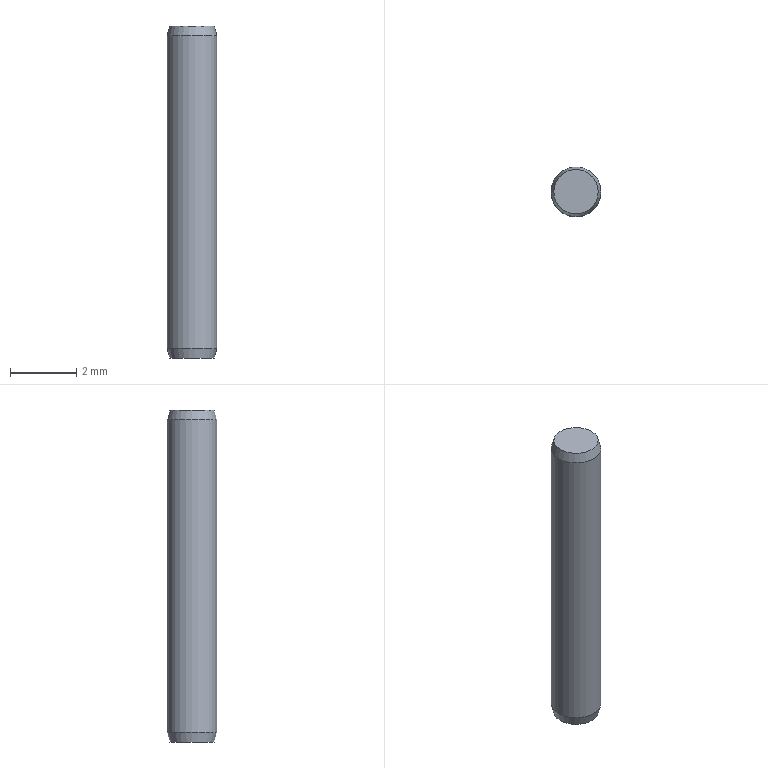Component | NX | GB-T119_1-2000_1_5X10 | 1 solid | 5 faces | box 1.5 x 1.5 x 10 mm | volume 18 mm3 | plane 2 | cone 2 | cylinder 1 | commonest cylinder face diameters 1.5 x1
STEP:
#1=CARTESIAN_POINT('',(0.,0.,0.));
#2=DIRECTION('',(0.,0.,1.));
#3=DIRECTION('',(1.,0.,0.));
#4=AXIS2_PLACEMENT_3D('',#1,#2,#3);
#5=CARTESIAN_POINT('',(-0.6696,65.,28.5));
#6=VERTEX_POINT('',#5);
#7=CARTESIAN_POINT('',(0.,65.,28.5));
#8=DIRECTION('',(0.,0.,-1.));
#9=DIRECTION('',(-1.,0.,0.));
#10=AXIS2_PLACEMENT_3D('',#7,#8,#9);
#11=CIRCLE('',#10,0.6696);
#12=CARTESIAN_POINT('',(0.,65.,28.5));
#13=DIRECTION('',(0.,0.,-1.));
#14=DIRECTION('',(-1.,0.,0.));
#15=AXIS2_PLACEMENT_3D('',#12,#13,#14);
#16=PLANE('',#15);
#17=CARTESIAN_POINT('',(0.,0.));
#18=DIRECTION('',(1.,0.));
#19=AXIS2_PLACEMENT_2D('',#17,#18);
#20=CIRCLE('',#19,0.6696);
#21=(GEOMETRIC_REPRESENTATION_CONTEXT(2)PARAMETRIC_REPRESENTATION_CONTEXT()REPRESENTATION_CONTEXT('',''));
#22=DEFINITIONAL_REPRESENTATION('',(#20),#21);
#23=PCURVE('',#16,#22);
#24=CARTESIAN_POINT('',(0.,65.,28.5));
#25=DIRECTION('',(0.,0.,1.));
#26=DIRECTION('',(1.,0.,0.));
#27=AXIS2_PLACEMENT_3D('',#24,#25,#26);
#28=CONICAL_SURFACE('',#27,0.6696,0.2618);
#29=CARTESIAN_POINT('',(9.425,0.));
#30=DIRECTION('',(-1.,0.));
#31=VECTOR('',#30,1.);
#32=LINE('',#29,#31);
#33=(GEOMETRIC_REPRESENTATION_CONTEXT(2)PARAMETRIC_REPRESENTATION_CONTEXT()REPRESENTATION_CONTEXT('',''));
#34=DEFINITIONAL_REPRESENTATION('',(#32),#33);
#35=PCURVE('',#28,#34);
#36=SURFACE_CURVE('',#11,(#23,#35),.PCURVE_S1.);
#37=EDGE_CURVE('',#6,#6,#36,.T.);
#38=ORIENTED_EDGE('',*,*,#37,.T.);
#39=EDGE_LOOP('',(#38));
#40=FACE_BOUND('',#39,.T.);
#41=ADVANCED_FACE('',(#40),#16,.T.);
#42=CARTESIAN_POINT('',(-0.75,65.,28.8));
#43=VERTEX_POINT('',#42);
#44=CARTESIAN_POINT('',(0.,65.,28.8));
#45=DIRECTION('',(0.,0.,-1.));
#46=DIRECTION('',(-1.,0.,0.));
#47=AXIS2_PLACEMENT_3D('',#44,#45,#46);
#48=CIRCLE('',#47,0.75);
#49=CARTESIAN_POINT('',(9.425,0.3));
#50=DIRECTION('',(-1.,0.));
#51=VECTOR('',#50,1.);
#52=LINE('',#49,#51);
#53=(GEOMETRIC_REPRESENTATION_CONTEXT(2)PARAMETRIC_REPRESENTATION_CONTEXT()REPRESENTATION_CONTEXT('',''));
#54=DEFINITIONAL_REPRESENTATION('',(#52),#53);
#55=PCURVE('',#28,#54);
#56=CARTESIAN_POINT('',(0.,65.,38.5));
#57=DIRECTION('',(0.,0.,-1.));
#58=DIRECTION('',(-1.,0.,0.));
#59=AXIS2_PLACEMENT_3D('',#56,#57,#58);
#60=CYLINDRICAL_SURFACE('',#59,0.75);
#61=CARTESIAN_POINT('',(0.,9.7));
#62=DIRECTION('',(1.,0.));
#63=VECTOR('',#62,1.);
#64=LINE('',#61,#63);
#65=(GEOMETRIC_REPRESENTATION_CONTEXT(2)PARAMETRIC_REPRESENTATION_CONTEXT()REPRESENTATION_CONTEXT('',''));
#66=DEFINITIONAL_REPRESENTATION('',(#64),#65);
#67=PCURVE('',#60,#66);
#68=SURFACE_CURVE('',#48,(#55,#67),.PCURVE_S1.);
#69=EDGE_CURVE('',#43,#43,#68,.T.);
#70=ORIENTED_EDGE('',*,*,#69,.T.);
#71=CARTESIAN_POINT('',(-0.6696,65.,28.5));
#72=CARTESIAN_POINT('',(-0.75,65.,28.8));
#73=B_SPLINE_CURVE_WITH_KNOTS('',1,(#71,#72),.UNSPECIFIED.,.F.,.F.,(2,2),(0.,0.3106),.PIECEWISE_BEZIER_KNOTS.);
#74=CARTESIAN_POINT('',(3.142,0.));
#75=DIRECTION('',(0.,1.));
#76=VECTOR('',#75,1.);
#77=LINE('',#74,#76);
#78=(GEOMETRIC_REPRESENTATION_CONTEXT(2)PARAMETRIC_REPRESENTATION_CONTEXT()REPRESENTATION_CONTEXT('',''));
#79=DEFINITIONAL_REPRESENTATION('',(#77),#78);
#80=PCURVE('',#28,#79);
#81=CARTESIAN_POINT('',(9.425,0.));
#82=DIRECTION('',(0.,1.));
#83=VECTOR('',#82,1.);
#84=LINE('',#81,#83);
#85=(GEOMETRIC_REPRESENTATION_CONTEXT(2)PARAMETRIC_REPRESENTATION_CONTEXT()REPRESENTATION_CONTEXT('',''));
#86=DEFINITIONAL_REPRESENTATION('',(#84),#85);
#87=PCURVE('',#28,#86);
#88=SEAM_CURVE('',#73,(#80,#87),.PCURVE_S1.);
#89=EDGE_CURVE('',#6,#43,#88,.T.);
#90=ORIENTED_EDGE('',*,*,#89,.F.);
#91=ORIENTED_EDGE('',*,*,#37,.F.);
#92=ORIENTED_EDGE('',*,*,#89,.T.);
#93=EDGE_LOOP('',(#70,#90,#91,#92));
#94=FACE_BOUND('',#93,.T.);
#95=ADVANCED_FACE('',(#94),#28,.T.);
#96=CARTESIAN_POINT('',(-0.75,65.,38.2));
#97=VERTEX_POINT('',#96);
#98=CARTESIAN_POINT('',(0.,65.,38.2));
#99=DIRECTION('',(0.,0.,-1.));
#100=DIRECTION('',(-1.,0.,0.));
#101=AXIS2_PLACEMENT_3D('',#98,#99,#100);
#102=CIRCLE('',#101,0.75);
#103=CARTESIAN_POINT('',(0.,0.3));
#104=DIRECTION('',(1.,0.));
#105=VECTOR('',#104,1.);
#106=LINE('',#103,#105);
#107=(GEOMETRIC_REPRESENTATION_CONTEXT(2)PARAMETRIC_REPRESENTATION_CONTEXT()REPRESENTATION_CONTEXT('',''));
#108=DEFINITIONAL_REPRESENTATION('',(#106),#107);
#109=PCURVE('',#60,#108);
#110=CARTESIAN_POINT('',(0.,65.,38.2));
#111=DIRECTION('',(0.,0.,-1.));
#112=DIRECTION('',(-1.,0.,0.));
#113=AXIS2_PLACEMENT_3D('',#110,#111,#112);
#114=CONICAL_SURFACE('',#113,0.75,0.2618);
#115=CARTESIAN_POINT('',(0.,0.));
#116=DIRECTION('',(1.,0.));
#117=VECTOR('',#116,1.);
#118=LINE('',#115,#117);
#119=(GEOMETRIC_REPRESENTATION_CONTEXT(2)PARAMETRIC_REPRESENTATION_CONTEXT()REPRESENTATION_CONTEXT('',''));
#120=DEFINITIONAL_REPRESENTATION('',(#118),#119);
#121=PCURVE('',#114,#120);
#122=SURFACE_CURVE('',#102,(#109,#121),.PCURVE_S1.);
#123=EDGE_CURVE('',#97,#97,#122,.T.);
#124=ORIENTED_EDGE('',*,*,#123,.T.);
#125=CARTESIAN_POINT('',(-0.75,65.,38.2));
#126=CARTESIAN_POINT('',(-0.75,65.,28.8));
#127=B_SPLINE_CURVE_WITH_KNOTS('',1,(#125,#126),.UNSPECIFIED.,.F.,.F.,(2,2),(0.3,9.7),.PIECEWISE_BEZIER_KNOTS.);
#128=CARTESIAN_POINT('',(6.283,0.));
#129=DIRECTION('',(0.,1.));
#130=VECTOR('',#129,1.);
#131=LINE('',#128,#130);
#132=(GEOMETRIC_REPRESENTATION_CONTEXT(2)PARAMETRIC_REPRESENTATION_CONTEXT()REPRESENTATION_CONTEXT('',''));
#133=DEFINITIONAL_REPRESENTATION('',(#131),#132);
#134=PCURVE('',#60,#133);
#135=CARTESIAN_POINT('',(0.,0.));
#136=DIRECTION('',(0.,1.));
#137=VECTOR('',#136,1.);
#138=LINE('',#135,#137);
#139=(GEOMETRIC_REPRESENTATION_CONTEXT(2)PARAMETRIC_REPRESENTATION_CONTEXT()REPRESENTATION_CONTEXT('',''));
#140=DEFINITIONAL_REPRESENTATION('',(#138),#139);
#141=PCURVE('',#60,#140);
#142=SEAM_CURVE('',#127,(#134,#141),.PCURVE_S1.);
#143=EDGE_CURVE('',#97,#43,#142,.T.);
#144=ORIENTED_EDGE('',*,*,#143,.T.);
#145=ORIENTED_EDGE('',*,*,#69,.F.);
#146=ORIENTED_EDGE('',*,*,#143,.F.);
#147=EDGE_LOOP('',(#124,#144,#145,#146));
#148=FACE_BOUND('',#147,.T.);
#149=ADVANCED_FACE('',(#148),#60,.T.);
#150=CARTESIAN_POINT('',(-0.6696,65.,38.5));
#151=VERTEX_POINT('',#150);
#152=CARTESIAN_POINT('',(0.,65.,38.5));
#153=DIRECTION('',(0.,0.,-1.));
#154=DIRECTION('',(-1.,0.,0.));
#155=AXIS2_PLACEMENT_3D('',#152,#153,#154);
#156=CIRCLE('',#155,0.6696);
#157=CARTESIAN_POINT('',(0.,-0.3));
#158=DIRECTION('',(1.,0.));
#159=VECTOR('',#158,1.);
#160=LINE('',#157,#159);
#161=(GEOMETRIC_REPRESENTATION_CONTEXT(2)PARAMETRIC_REPRESENTATION_CONTEXT()REPRESENTATION_CONTEXT('',''));
#162=DEFINITIONAL_REPRESENTATION('',(#160),#161);
#163=PCURVE('',#114,#162);
#164=CARTESIAN_POINT('',(0.6696,65.,38.5));
#165=DIRECTION('',(0.,0.,1.));
#166=DIRECTION('',(1.,0.,0.));
#167=AXIS2_PLACEMENT_3D('',#164,#165,#166);
#168=PLANE('',#167);
#169=CARTESIAN_POINT('',(-1.339,0.));
#170=CARTESIAN_POINT('',(-1.339,1.16));
#171=CARTESIAN_POINT('',(-0.3348,0.5799));
#172=CARTESIAN_POINT('',(0.6696,0.));
#173=CARTESIAN_POINT('',(-0.3348,-0.5799));
#174=CARTESIAN_POINT('',(-1.339,-1.16));
#175=CARTESIAN_POINT('',(-1.339,0.));
#176=(BOUNDED_CURVE()B_SPLINE_CURVE(2,(#169,#170,#171,#172,#173,#174,#175),.UNSPECIFIED.,.T.,.F.)B_SPLINE_CURVE_WITH_KNOTS((1,2,2,2,2,1),(-2.094,0.,2.094,4.189,6.283,8.378),.UNSPECIFIED.)CURVE()GEOMETRIC_REPRESENTATION_ITEM()RATIONAL_B_SPLINE_CURVE((1.,0.5,1.,0.5,1.,0.5,1.))REPRESENTATION_ITEM(''));
#177=(GEOMETRIC_REPRESENTATION_CONTEXT(2)PARAMETRIC_REPRESENTATION_CONTEXT()REPRESENTATION_CONTEXT('',''));
#178=DEFINITIONAL_REPRESENTATION('',(#176),#177);
#179=PCURVE('',#168,#178);
#180=SURFACE_CURVE('',#156,(#163,#179),.PCURVE_S1.);
#181=EDGE_CURVE('',#151,#151,#180,.T.);
#182=ORIENTED_EDGE('',*,*,#181,.T.);
#183=CARTESIAN_POINT('',(-0.6696,65.,38.5));
#184=CARTESIAN_POINT('',(-0.75,65.,38.2));
#185=B_SPLINE_CURVE_WITH_KNOTS('',1,(#183,#184),.UNSPECIFIED.,.F.,.F.,(2,2),(-0.3106,0.),.PIECEWISE_BEZIER_KNOTS.);
#186=CARTESIAN_POINT('',(6.283,0.));
#187=DIRECTION('',(0.,1.));
#188=VECTOR('',#187,1.);
#189=LINE('',#186,#188);
#190=(GEOMETRIC_REPRESENTATION_CONTEXT(2)PARAMETRIC_REPRESENTATION_CONTEXT()REPRESENTATION_CONTEXT('',''));
#191=DEFINITIONAL_REPRESENTATION('',(#189),#190);
#192=PCURVE('',#114,#191);
#193=CARTESIAN_POINT('',(0.,0.));
#194=DIRECTION('',(0.,1.));
#195=VECTOR('',#194,1.);
#196=LINE('',#193,#195);
#197=(GEOMETRIC_REPRESENTATION_CONTEXT(2)PARAMETRIC_REPRESENTATION_CONTEXT()REPRESENTATION_CONTEXT('',''));
#198=DEFINITIONAL_REPRESENTATION('',(#196),#197);
#199=PCURVE('',#114,#198);
#200=SEAM_CURVE('',#185,(#192,#199),.PCURVE_S1.);
#201=EDGE_CURVE('',#151,#97,#200,.T.);
#202=ORIENTED_EDGE('',*,*,#201,.T.);
#203=ORIENTED_EDGE('',*,*,#123,.F.);
#204=ORIENTED_EDGE('',*,*,#201,.F.);
#205=EDGE_LOOP('',(#182,#202,#203,#204));
#206=FACE_BOUND('',#205,.T.);
#207=ADVANCED_FACE('',(#206),#114,.T.);
#208=ORIENTED_EDGE('',*,*,#181,.F.);
#209=EDGE_LOOP('',(#208));
#210=FACE_BOUND('',#209,.T.);
#211=ADVANCED_FACE('',(#210),#168,.T.);
#212=CLOSED_SHELL('',(#41,#95,#149,#207,#211));
#213=MANIFOLD_SOLID_BREP('',#212);
#214=(LENGTH_UNIT()NAMED_UNIT(*)SI_UNIT(.MILLI.,.METRE.));
#215=UNCERTAINTY_MEASURE_WITH_UNIT(LENGTH_MEASURE(0.00001),#214,'','');
#216=(NAMED_UNIT(*)PLANE_ANGLE_UNIT()SI_UNIT($,.RADIAN.));
#217=(NAMED_UNIT(*)SI_UNIT($,.STERADIAN.)SOLID_ANGLE_UNIT());
#218=(GEOMETRIC_REPRESENTATION_CONTEXT(3)GLOBAL_UNCERTAINTY_ASSIGNED_CONTEXT((#215))GLOBAL_UNIT_ASSIGNED_CONTEXT((#214,#216,#217))REPRESENTATION_CONTEXT('',''));
#219=ADVANCED_BREP_SHAPE_REPRESENTATION('',(#4,#213),#218);